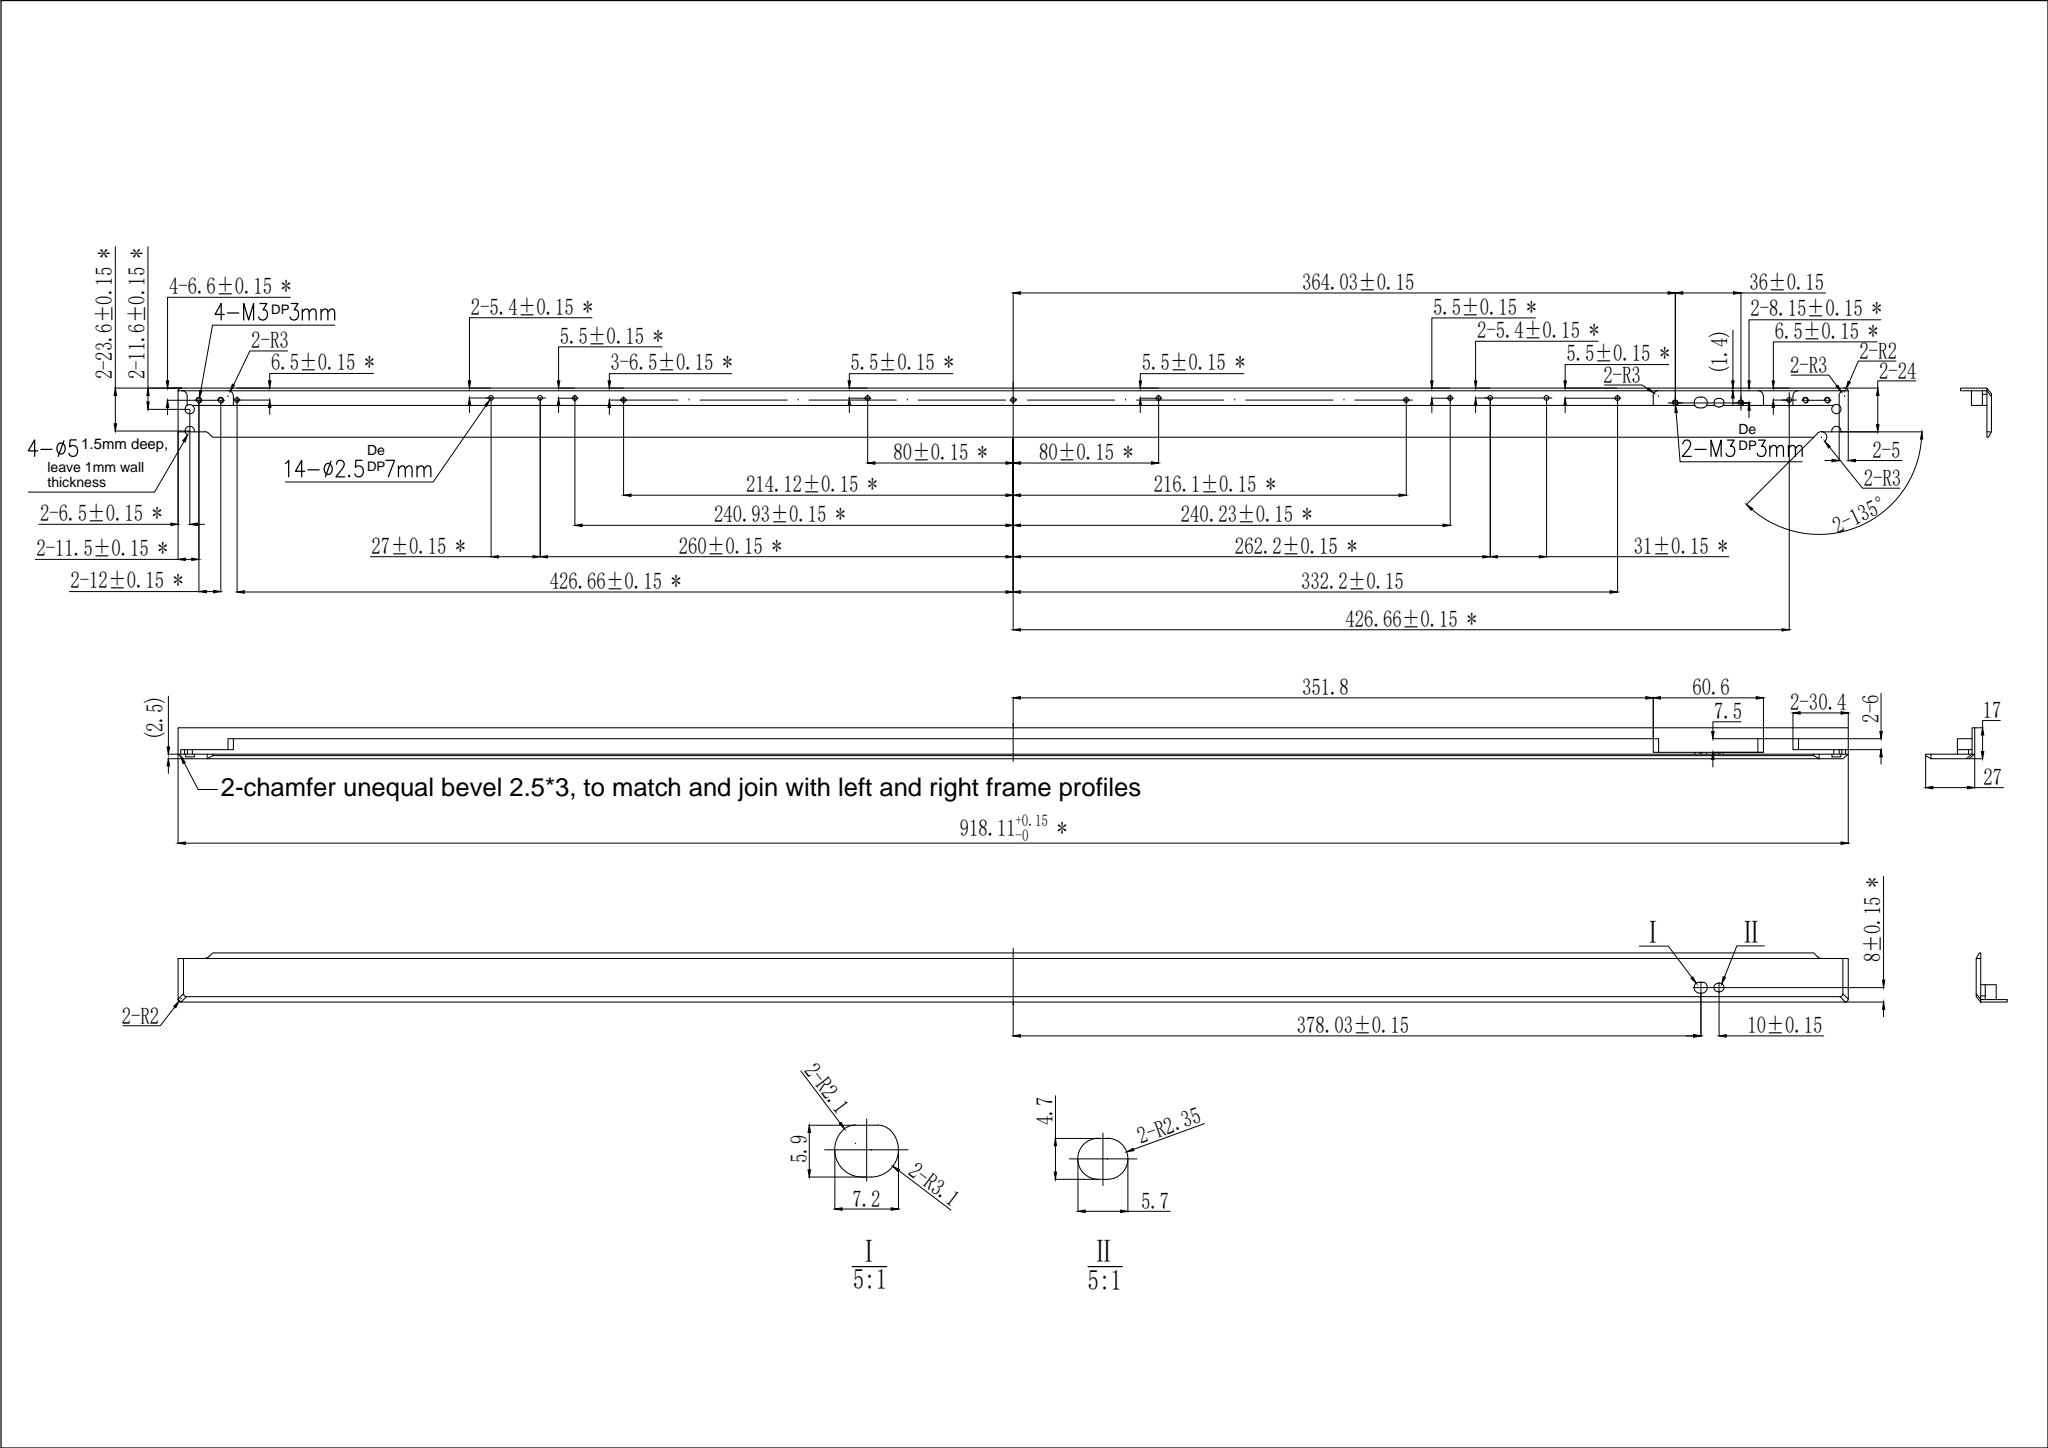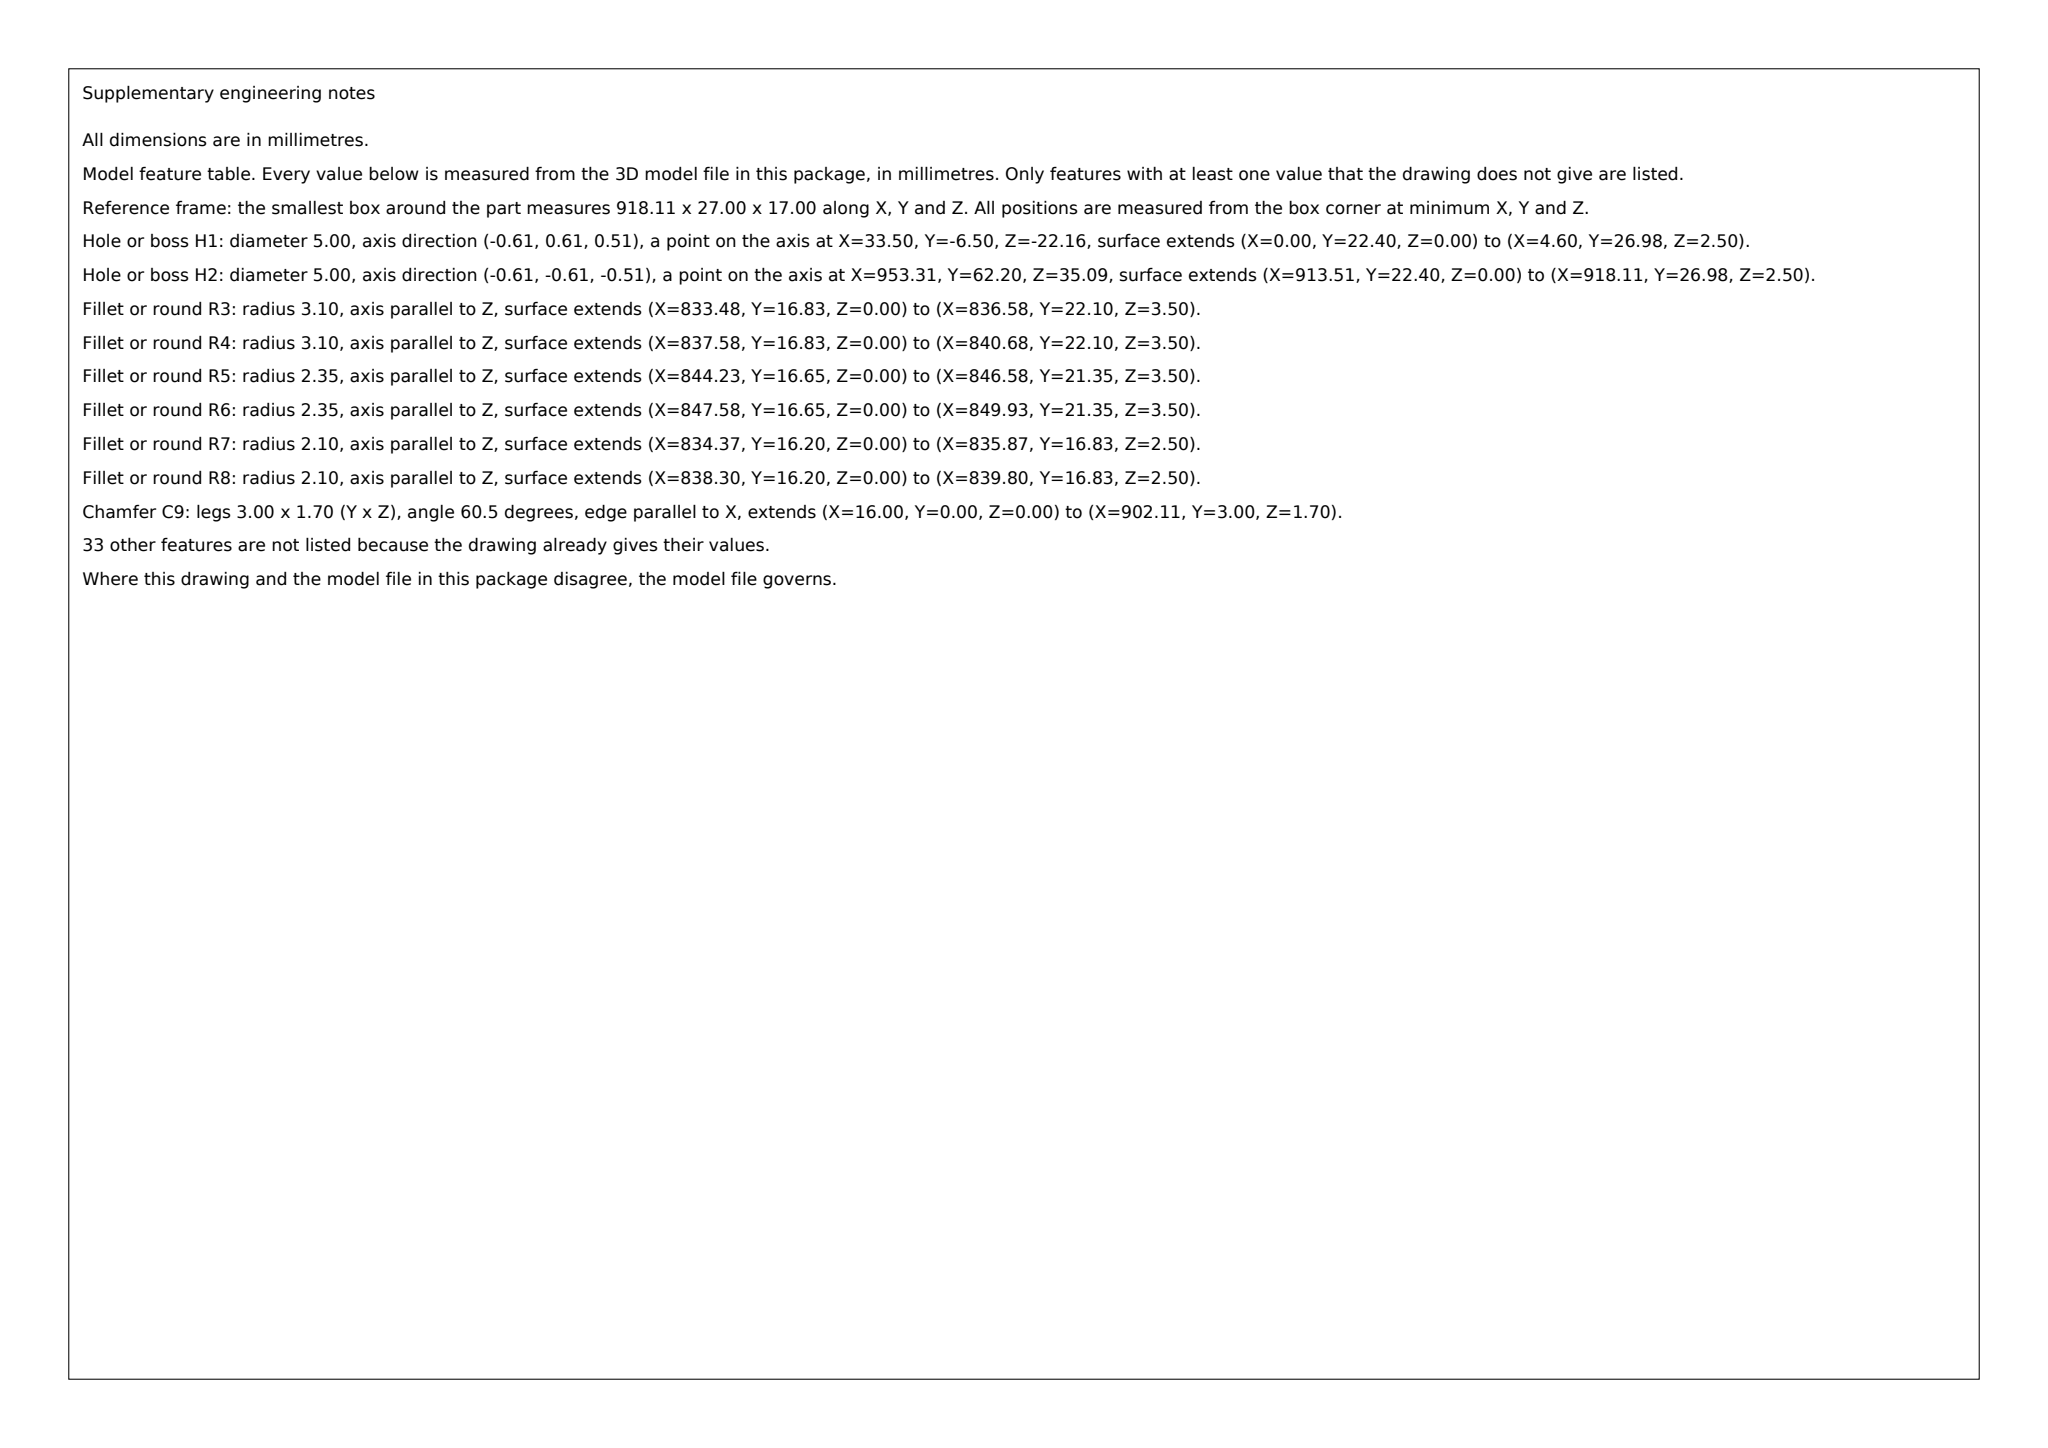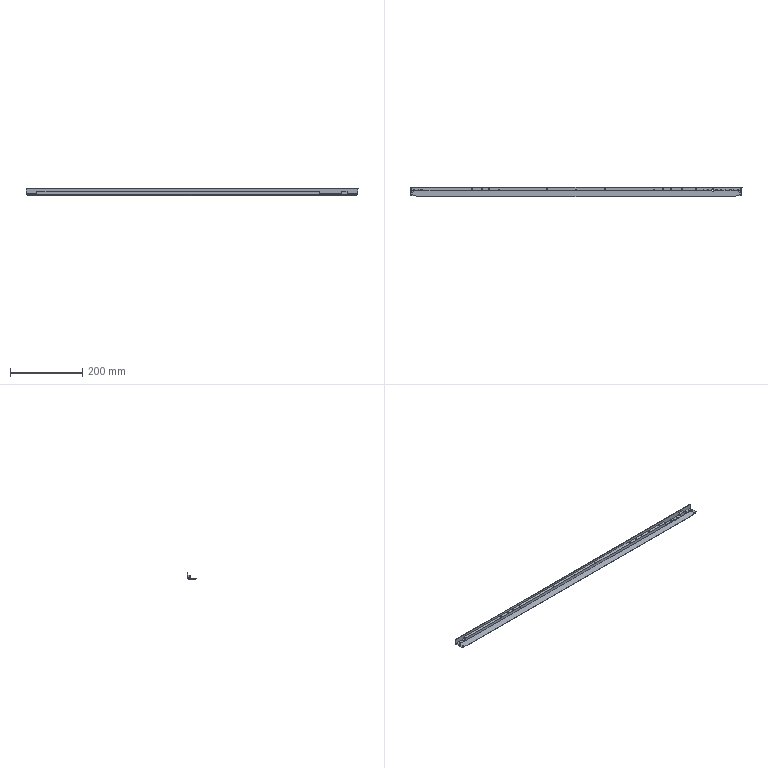Part | SolidWorks | mm | 1 solid | 122 faces | box 918.11 x 27 x 17 mm | volume 130029 mm3 | cylinder 64 | plane 58 | commonest cylinder face diameters 2.5 x40 5 x12 4 x4 4.7 x3 6.2 x3 4.2 x2